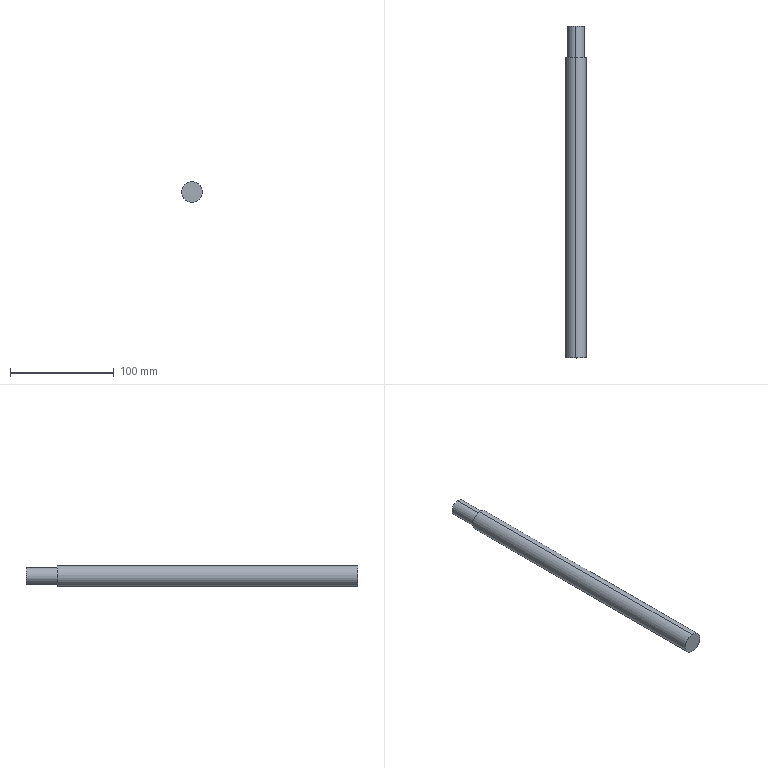Component | SolidWorks | ColumnCylinderPistonRod-1 | 1 solid | 7 faces | box 20 x 320 x 20 mm | volume 97138 mm3 | cylinder 4 | plane 3 | commonest cylinder face diameters 16 x2 20 x2
build123d program:
from build123d import *

# Parameters (mm, degrees)
SKETCH1_R           = 10
BOSS_EXTRUDE1_DEPTH = 290
SKETCH2_R           = 8
BOSS_EXTRUDE2_DEPTH = 30


with BuildPart() as part:
    # Sketch1 → Boss-Extrude1 (new body)
    with BuildSketch(Plane(origin=(0, 0, 0), x_dir=(1, 0, 0), z_dir=(0, 1, 0))):
        with Locations(Location((0, 0, 0), (0, 0, 270))):
            Circle(SKETCH1_R)
    extrude(amount=BOSS_EXTRUDE1_DEPTH)

    # Sketch2 → Boss-Extrude2 (add)
    with BuildSketch(Plane(origin=(0, 290, 0), x_dir=(1, 0, 0), z_dir=(0, 1, 0))):
        with Locations(Location((0, 0, 0), (0, 0, 270))):
            Circle(SKETCH2_R)
    extrude(amount=BOSS_EXTRUDE2_DEPTH)


solid = part.part

# Placed as in the assembly
solid = solid.moved(Location((-87.309, 476.583, 566.392), (0, 0, 0)))
STEP:
#1=COLOUR_RGB('',0.7922,0.8196,0.9333);
#2=FILL_AREA_STYLE_COLOUR('',#1);
#3=FILL_AREA_STYLE('',(#2));
#4=SURFACE_STYLE_FILL_AREA(#3);
#5=SURFACE_SIDE_STYLE('',(#4));
#6=SURFACE_STYLE_USAGE(.BOTH.,#5);
#7=PRESENTATION_STYLE_ASSIGNMENT((#6));
#8=CARTESIAN_POINT('',(-3.459,31.362,22.613));
#9=VERTEX_POINT('',#8);
#10=CARTESIAN_POINT('',(-3.416,31.362,21.985));
#11=VERTEX_POINT('',#10);
#12=CARTESIAN_POINT('',(-3.437,31.362,22.299));
#13=DIRECTION('',(0.,1.,0.));
#14=DIRECTION('',(-0.06811,0.,0.9977));
#15=AXIS2_PLACEMENT_3D('',#12,#13,#14);
#16=CIRCLE('',#15,0.315);
#17=EDGE_CURVE('',#9,#11,#16,.T.);
#18=ORIENTED_EDGE('',*,*,#17,.F.);
#19=CARTESIAN_POINT('',(-3.459,30.18,22.613));
#20=VERTEX_POINT('',#19);
#21=CARTESIAN_POINT('',(-3.459,31.362,22.613));
#22=DIRECTION('',(0.,-1.,0.));
#23=VECTOR('',#22,39.37);
#24=LINE('',#21,#23);
#25=EDGE_CURVE('',#9,#20,#24,.T.);
#26=ORIENTED_EDGE('',*,*,#25,.T.);
#27=CARTESIAN_POINT('',(-3.416,30.18,21.985));
#28=VERTEX_POINT('',#27);
#29=CARTESIAN_POINT('',(-3.437,30.18,22.299));
#30=DIRECTION('',(0.,1.,0.));
#31=DIRECTION('',(-0.06811,0.,0.9977));
#32=AXIS2_PLACEMENT_3D('',#29,#30,#31);
#33=CIRCLE('',#32,0.315);
#34=EDGE_CURVE('',#20,#28,#33,.T.);
#35=ORIENTED_EDGE('',*,*,#34,.T.);
#36=CARTESIAN_POINT('',(-3.416,31.362,21.985));
#37=DIRECTION('',(0.,-1.,0.));
#38=VECTOR('',#37,39.37);
#39=LINE('',#36,#38);
#40=EDGE_CURVE('',#11,#28,#39,.T.);
#41=ORIENTED_EDGE('',*,*,#40,.F.);
#42=EDGE_LOOP('',(#18,#26,#35,#41));
#43=FACE_OUTER_BOUND('',#42,.T.);
#44=CARTESIAN_POINT('',(-3.437,31.362,22.299));
#45=DIRECTION('',(0.,-1.,0.));
#46=DIRECTION('',(0.06811,0.,-0.9977));
#47=AXIS2_PLACEMENT_3D('',#44,#45,#46);
#48=CYLINDRICAL_SURFACE('',#47,0.315);
#49=ADVANCED_FACE('',(#43),#48,.T.);
#50=CARTESIAN_POINT('',(-3.464,30.18,22.692));
#51=VERTEX_POINT('',#50);
#52=CARTESIAN_POINT('',(-3.411,30.18,21.906));
#53=VERTEX_POINT('',#52);
#54=CARTESIAN_POINT('',(-3.437,30.18,22.299));
#55=DIRECTION('',(0.,1.,0.));
#56=DIRECTION('',(-0.06811,0.,0.9977));
#57=AXIS2_PLACEMENT_3D('',#54,#55,#56);
#58=CIRCLE('',#57,0.3937);
#59=EDGE_CURVE('',#51,#53,#58,.T.);
#60=ORIENTED_EDGE('',*,*,#59,.F.);
#61=CARTESIAN_POINT('',(-3.464,18.763,22.692));
#62=VERTEX_POINT('',#61);
#63=CARTESIAN_POINT('',(-3.464,30.18,22.692));
#64=DIRECTION('',(0.,-1.,0.));
#65=VECTOR('',#64,39.37);
#66=LINE('',#63,#65);
#67=EDGE_CURVE('',#51,#62,#66,.T.);
#68=ORIENTED_EDGE('',*,*,#67,.T.);
#69=CARTESIAN_POINT('',(-3.411,18.763,21.906));
#70=VERTEX_POINT('',#69);
#71=CARTESIAN_POINT('',(-3.437,18.763,22.299));
#72=DIRECTION('',(0.,1.,0.));
#73=DIRECTION('',(-0.06811,0.,0.9977));
#74=AXIS2_PLACEMENT_3D('',#71,#72,#73);
#75=CIRCLE('',#74,0.3937);
#76=EDGE_CURVE('',#62,#70,#75,.T.);
#77=ORIENTED_EDGE('',*,*,#76,.T.);
#78=CARTESIAN_POINT('',(-3.411,30.18,21.906));
#79=DIRECTION('',(0.,-1.,0.));
#80=VECTOR('',#79,39.37);
#81=LINE('',#78,#80);
#82=EDGE_CURVE('',#53,#70,#81,.T.);
#83=ORIENTED_EDGE('',*,*,#82,.F.);
#84=EDGE_LOOP('',(#60,#68,#77,#83));
#85=FACE_OUTER_BOUND('',#84,.T.);
#86=CARTESIAN_POINT('',(-3.437,30.18,22.299));
#87=DIRECTION('',(0.,-1.,0.));
#88=DIRECTION('',(0.06811,0.,-0.9977));
#89=AXIS2_PLACEMENT_3D('',#86,#87,#88);
#90=CYLINDRICAL_SURFACE('',#89,0.3937);
#91=ADVANCED_FACE('',(#85),#90,.T.);
#92=ORIENTED_EDGE('',*,*,#67,.F.);
#93=CARTESIAN_POINT('',(-3.437,30.18,22.299));
#94=DIRECTION('',(0.,1.,0.));
#95=DIRECTION('',(-0.06811,0.,0.9977));
#96=AXIS2_PLACEMENT_3D('',#93,#94,#95);
#97=CIRCLE('',#96,0.3937);
#98=EDGE_CURVE('',#53,#51,#97,.T.);
#99=ORIENTED_EDGE('',*,*,#98,.F.);
#100=ORIENTED_EDGE('',*,*,#82,.T.);
#101=CARTESIAN_POINT('',(-3.437,18.763,22.299));
#102=DIRECTION('',(0.,1.,0.));
#103=DIRECTION('',(-0.06811,0.,0.9977));
#104=AXIS2_PLACEMENT_3D('',#101,#102,#103);
#105=CIRCLE('',#104,0.3937);
#106=EDGE_CURVE('',#70,#62,#105,.T.);
#107=ORIENTED_EDGE('',*,*,#106,.T.);
#108=EDGE_LOOP('',(#92,#99,#100,#107));
#109=FACE_OUTER_BOUND('',#108,.T.);
#110=CARTESIAN_POINT('',(-3.437,30.18,22.299));
#111=DIRECTION('',(0.,-1.,0.));
#112=DIRECTION('',(0.06811,0.,-0.9977));
#113=AXIS2_PLACEMENT_3D('',#110,#111,#112);
#114=CYLINDRICAL_SURFACE('',#113,0.3937);
#115=ADVANCED_FACE('',(#109),#114,.T.);
#116=CARTESIAN_POINT('',(-3.437,30.18,22.299));
#117=DIRECTION('',(0.,1.,0.));
#118=DIRECTION('',(-0.06811,0.,0.9977));
#119=AXIS2_PLACEMENT_3D('',#116,#117,#118);
#120=CIRCLE('',#119,0.315);
#121=EDGE_CURVE('',#28,#20,#120,.T.);
#122=ORIENTED_EDGE('',*,*,#121,.F.);
#123=ORIENTED_EDGE('',*,*,#34,.F.);
#124=EDGE_LOOP('',(#122,#123));
#125=FACE_BOUND('',#124,.T.);
#126=ORIENTED_EDGE('',*,*,#98,.T.);
#127=ORIENTED_EDGE('',*,*,#59,.T.);
#128=EDGE_LOOP('',(#126,#127));
#129=FACE_OUTER_BOUND('',#128,.T.);
#130=CARTESIAN_POINT('',(-3.437,30.18,22.299));
#131=DIRECTION('',(0.,1.,0.));
#132=DIRECTION('',(-0.06811,0.,0.9977));
#133=AXIS2_PLACEMENT_3D('',#130,#131,#132);
#134=PLANE('',#133);
#135=ADVANCED_FACE('',(#125,#129),#134,.T.);
#136=ORIENTED_EDGE('',*,*,#106,.F.);
#137=ORIENTED_EDGE('',*,*,#76,.F.);
#138=EDGE_LOOP('',(#136,#137));
#139=FACE_OUTER_BOUND('',#138,.T.);
#140=CARTESIAN_POINT('',(-3.437,18.763,22.299));
#141=DIRECTION('',(0.,1.,0.));
#142=DIRECTION('',(-0.06811,0.,0.9977));
#143=AXIS2_PLACEMENT_3D('',#140,#141,#142);
#144=PLANE('',#143);
#145=ADVANCED_FACE('',(#139),#144,.F.);
#146=ORIENTED_EDGE('',*,*,#25,.F.);
#147=CARTESIAN_POINT('',(-3.437,31.362,22.299));
#148=DIRECTION('',(0.,1.,0.));
#149=DIRECTION('',(-0.06811,0.,0.9977));
#150=AXIS2_PLACEMENT_3D('',#147,#148,#149);
#151=CIRCLE('',#150,0.315);
#152=EDGE_CURVE('',#11,#9,#151,.T.);
#153=ORIENTED_EDGE('',*,*,#152,.F.);
#154=ORIENTED_EDGE('',*,*,#40,.T.);
#155=ORIENTED_EDGE('',*,*,#121,.T.);
#156=EDGE_LOOP('',(#146,#153,#154,#155));
#157=FACE_OUTER_BOUND('',#156,.T.);
#158=CARTESIAN_POINT('',(-3.437,31.362,22.299));
#159=DIRECTION('',(0.,-1.,0.));
#160=DIRECTION('',(0.06811,0.,-0.9977));
#161=AXIS2_PLACEMENT_3D('',#158,#159,#160);
#162=CYLINDRICAL_SURFACE('',#161,0.315);
#163=ADVANCED_FACE('',(#157),#162,.T.);
#164=ORIENTED_EDGE('',*,*,#152,.T.);
#165=ORIENTED_EDGE('',*,*,#17,.T.);
#166=EDGE_LOOP('',(#164,#165));
#167=FACE_OUTER_BOUND('',#166,.T.);
#168=CARTESIAN_POINT('',(-3.437,31.362,22.299));
#169=DIRECTION('',(0.,1.,0.));
#170=DIRECTION('',(-0.06811,0.,0.9977));
#171=AXIS2_PLACEMENT_3D('',#168,#169,#170);
#172=PLANE('',#171);
#173=ADVANCED_FACE('',(#167),#172,.T.);
#174=CLOSED_SHELL('',(#49,#91,#115,#135,#145,#163,#173));
#175=MANIFOLD_SOLID_BREP('',#174);
#176=STYLED_ITEM('',(#7),#175);
#177=PRESENTATION_LAYER_ASSIGNMENT('','',(#176));
#178=(LENGTH_UNIT()NAMED_UNIT(*)SI_UNIT($,.METRE.));
#179=LENGTH_MEASURE_WITH_UNIT(LENGTH_MEASURE(0.0254),#178);
#180=DIMENSIONAL_EXPONENTS(1.,0.,0.,0.,0.,0.,0.);
#181=(CONVERSION_BASED_UNIT('',#179)LENGTH_UNIT()NAMED_UNIT(#180));
#182=UNCERTAINTY_MEASURE_WITH_UNIT(LENGTH_MEASURE(0.00001),#181,'','');
#183=(NAMED_UNIT(*)PLANE_ANGLE_UNIT()SI_UNIT($,.RADIAN.));
#184=(NAMED_UNIT(*)SI_UNIT($,.STERADIAN.)SOLID_ANGLE_UNIT());
#185=(GEOMETRIC_REPRESENTATION_CONTEXT(3)GLOBAL_UNCERTAINTY_ASSIGNED_CONTEXT((#182))GLOBAL_UNIT_ASSIGNED_CONTEXT((#181,#183,#184))REPRESENTATION_CONTEXT('',''));
#186=MECHANICAL_DESIGN_GEOMETRIC_PRESENTATION_REPRESENTATION('',(#176),#185);
#187=CARTESIAN_POINT('',(0.,0.,0.));
#188=DIRECTION('',(0.,0.,1.));
#189=DIRECTION('',(1.,0.,0.));
#190=AXIS2_PLACEMENT_3D('',#187,#188,#189);
#191=(LENGTH_UNIT()NAMED_UNIT(*)SI_UNIT($,.METRE.));
#192=LENGTH_MEASURE_WITH_UNIT(LENGTH_MEASURE(0.0254),#191);
#193=DIMENSIONAL_EXPONENTS(1.,0.,0.,0.,0.,0.,0.);
#194=(CONVERSION_BASED_UNIT('',#192)LENGTH_UNIT()NAMED_UNIT(#193));
#195=UNCERTAINTY_MEASURE_WITH_UNIT(LENGTH_MEASURE(0.00001),#194,'','');
#196=(NAMED_UNIT(*)PLANE_ANGLE_UNIT()SI_UNIT($,.RADIAN.));
#197=(NAMED_UNIT(*)SI_UNIT($,.STERADIAN.)SOLID_ANGLE_UNIT());
#198=(GEOMETRIC_REPRESENTATION_CONTEXT(3)GLOBAL_UNCERTAINTY_ASSIGNED_CONTEXT((#195))GLOBAL_UNIT_ASSIGNED_CONTEXT((#194,#196,#197))REPRESENTATION_CONTEXT('',''));
#199=ADVANCED_BREP_SHAPE_REPRESENTATION('',(#175,#190),#198);